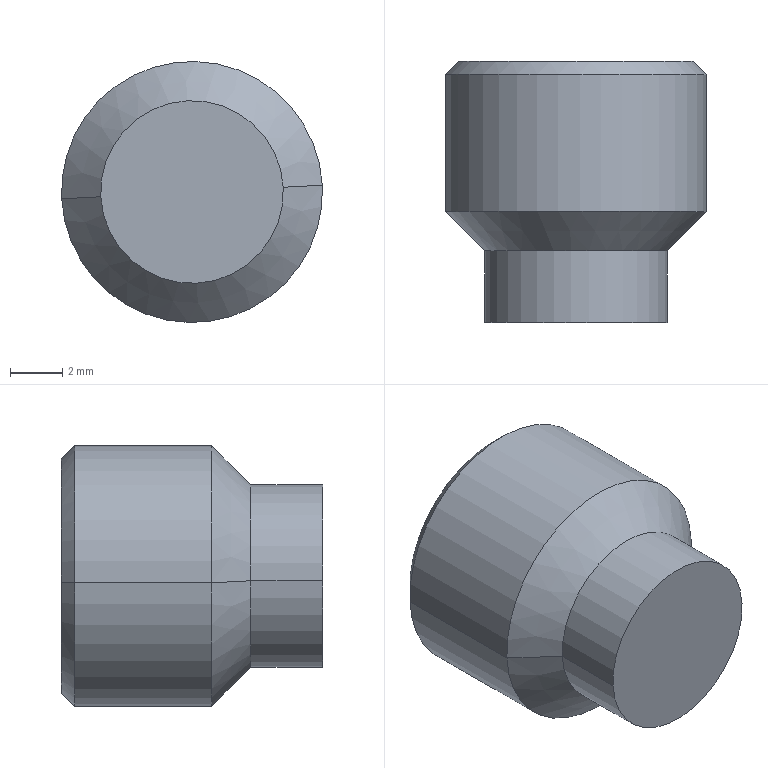Component | SolidWorks | 4-12-12ClampingAxisAssembly-1_4-12-9HeadlessSetScrew-D10-1 | 1 solid | 30 faces | box 10 x 10 x 10 mm | volume 559 mm3 | plane 18 | cone 6 | cylinder 6 | commonest cylinder face diameters 7 x2 5 x2 10 x2
build123d program:
from build123d import *

# Parameters (mm, degrees)
SKETCH1_R            = 2.463
BASE_EXTRUDE_DEPTH   = 20
LPATTERN1_COUNT      = 8
LPATTERN1_PITCH      = 1
SKETCH7_W            = 5
SKETCH7_H            = 6
CUT_EXTRUDE2_DEPTH   = 3
SKETCH4_2_R          = 7.956
CUT_EXTRUDE2_2_DEPTH = 27
SKETCH5_2_R          = 5
EXTRUDE1_DEPTH       = 4
CHAMFER1_SIZE        = 0.5


with BuildPart() as part:
    # Sketch1 → Base-Extrude (new body)
    with BuildSketch(Plane.XY):
        Circle(SKETCH1_R)
    extrude(amount=BASE_EXTRUDE_DEPTH)

    # Boss-Sweep1: sweep along a path in Sketch4
    with BuildLine(Plane(origin=(0, 0, 0.5), x_dir=(-1, 0, 0), z_dir=(0, 0, -1))) as boss_sweep1_path:
        CenterArc((0, 0), 2.463, 0, 360)
    # Sketch2 → Boss-Sweep1 (sweep)
    with BuildSketch(Plane(origin=(0, 0, 0), x_dir=(1, 0, 0), z_dir=(0, 1, 0))):
        Polygon((2.463, 0), (3, -0.3103), (3, -0.4353), (2.463, -0.7457), align=None)
    boss_sweep1 = sweep(path=boss_sweep1_path.line)

    # LPattern1: Boss-Sweep1 ×8
    with Locations(*[(0, 0, i * LPATTERN1_PITCH) for i in range(1, LPATTERN1_COUNT)]):
        add(boss_sweep1)

    # Sketch7 → Boss-Revolve2 (revolve)
    with BuildSketch(Plane(origin=(0, 0, 0), x_dir=(1, 0, 0), z_dir=(0, 1, 0))):
        with Locations((2.5, -23)):
            Rectangle(SKETCH7_W, SKETCH7_H)
    revolve(axis=Axis((0, 0, 0), (0, 0, 1)))

    # Sketch8 → Cut-Extrude2 (cut)
    with BuildSketch(Plane.XY.offset(26)):
        Polygon((-1.417, 2.5), (1.417, 2.5), (2.86, 0), (1.417, -2.5), (-1.417, -2.5), (-2.86, 0), align=None)
    extrude(amount=-CUT_EXTRUDE2_DEPTH, mode=Mode.SUBTRACT)

    # Sketch9 → Cut-Revolve1 (revolve, cut)
    with BuildSketch(Plane(origin=(0, 0, 0), x_dir=(1, 0, 0), z_dir=(0, 1, 0))):
        Polygon((0, -23), (2.5, -23), (2.5, -22.4), (0, -21.73), align=None)
    revolve(axis=Axis((0, 0, 0), (0, 0, 1)), mode=Mode.SUBTRACT)

    # Sketch4_2 → Cut-Extrude2_2 (cut)
    with BuildSketch(Plane(origin=(0, 0, 17.25), x_dir=(-1, 0, 0), z_dir=(0, 0, -1))):
        Circle(SKETCH4_2_R)
    extrude(amount=CUT_EXTRUDE2_2_DEPTH, mode=Mode.SUBTRACT)

    # Sketch5_2 → Extrude1 (add)
    with BuildSketch(Plane(origin=(0, 0, 20), x_dir=(-1, 0, 0), z_dir=(0, 0, -1))):
        Circle(SKETCH5_2_R)
    extrude(amount=EXTRUDE1_DEPTH)

    # Sketch7_2 → Cut-Revolve1_2 (revolve, cut)
    with BuildSketch(Plane(origin=(0, 0, 0), x_dir=(1, 0, 0), z_dir=(0, 1, 0)), mode=Mode.PRIVATE) as cut_revolve1_2_sk:
        Polygon((3.5, -16), (3.5, -18.75), (5, -20.25), (5, -16), align=None)
    revolve(cut_revolve1_2_sk.sketch.rotate(Axis((0, 0, 26), (0, 0, -1)), 180), axis=Axis((0, 0, 26), (0, 0, -1)), mode=Mode.SUBTRACT)

    # Chamfer1
    chamfer1_edges = [part.edges().sort_by_distance(p)[0] for p in [
        (-5, 0, 26),
    ]]
    chamfer(chamfer1_edges, length=CHAMFER1_SIZE)


solid = part.part

# Placed as in the assembly
solid = solid.moved(Location((-19.809, 9.85, 0), (-90, 0, 177)))
STEP:
#1=COLOUR_RGB('',0.7922,0.8196,0.9333);
#2=FILL_AREA_STYLE_COLOUR('',#1);
#3=FILL_AREA_STYLE('',(#2));
#4=SURFACE_STYLE_FILL_AREA(#3);
#5=SURFACE_SIDE_STYLE('',(#4));
#6=SURFACE_STYLE_USAGE(.BOTH.,#5);
#7=PRESENTATION_STYLE_ASSIGNMENT((#6));
#8=CARTESIAN_POINT('',(-0.603,1.411,0.009272));
#9=VERTEX_POINT('',#8);
#10=CARTESIAN_POINT('',(-0.9568,1.411,-0.009272));
#11=VERTEX_POINT('',#10);
#12=CARTESIAN_POINT('',(-0.7799,1.411,0.));
#13=DIRECTION('',(-0.,1.,-0.));
#14=DIRECTION('',(0.9986,0.,0.05234));
#15=AXIS2_PLACEMENT_3D('',#12,#13,#14);
#16=CIRCLE('',#15,0.1772);
#17=EDGE_CURVE('',#9,#11,#16,.T.);
#18=ORIENTED_EDGE('',*,*,#17,.F.);
#19=CARTESIAN_POINT('',(-0.5833,1.392,0.0103));
#20=VERTEX_POINT('',#19);
#21=CARTESIAN_POINT('',(-0.5833,1.392,0.0103));
#22=DIRECTION('',(0.7061,-0.7071,0.03701));
#23=VECTOR('',#22,39.37);
#24=LINE('',#21,#23);
#25=EDGE_CURVE('',#9,#20,#24,.T.);
#26=ORIENTED_EDGE('',*,*,#25,.T.);
#27=CARTESIAN_POINT('',(-0.9765,1.392,-0.0103));
#28=VERTEX_POINT('',#27);
#29=CARTESIAN_POINT('',(-0.7799,1.392,0.));
#30=DIRECTION('',(0.,-1.,0.));
#31=DIRECTION('',(0.9986,0.,0.05234));
#32=AXIS2_PLACEMENT_3D('',#29,#30,#31);
#33=CIRCLE('',#32,0.1969);
#34=EDGE_CURVE('',#28,#20,#33,.T.);
#35=ORIENTED_EDGE('',*,*,#34,.F.);
#36=CARTESIAN_POINT('',(-0.9765,1.392,-0.0103));
#37=DIRECTION('',(-0.7061,-0.7071,-0.03701));
#38=VECTOR('',#37,39.37);
#39=LINE('',#36,#38);
#40=EDGE_CURVE('',#11,#28,#39,.T.);
#41=ORIENTED_EDGE('',*,*,#40,.F.);
#42=EDGE_LOOP('',(#18,#26,#35,#41));
#43=FACE_OUTER_BOUND('',#42,.T.);
#44=CARTESIAN_POINT('',(-0.7799,1.392,0.));
#45=DIRECTION('',(0.,-1.,0.));
#46=DIRECTION('',(-0.9986,0.,-0.05234));
#47=AXIS2_PLACEMENT_3D('',#44,#45,#46);
#48=CONICAL_SURFACE('',#47,0.1969,0.7854);
#49=ADVANCED_FACE('',(#43),#48,.T.);
#50=CARTESIAN_POINT('',(-0.6423,1.018,0.007212));
#51=VERTEX_POINT('',#50);
#52=CARTESIAN_POINT('',(-0.9175,1.018,-0.007212));
#53=VERTEX_POINT('',#52);
#54=CARTESIAN_POINT('',(-0.7799,1.018,0.));
#55=DIRECTION('',(-0.,1.,-0.));
#56=DIRECTION('',(0.9986,0.,0.05234));
#57=AXIS2_PLACEMENT_3D('',#54,#55,#56);
#58=CIRCLE('',#57,0.1378);
#59=EDGE_CURVE('',#51,#53,#58,.T.);
#60=ORIENTED_EDGE('',*,*,#59,.T.);
#61=CARTESIAN_POINT('',(-0.9175,1.126,-0.007212));
#62=VERTEX_POINT('',#61);
#63=CARTESIAN_POINT('',(-0.9175,1.411,-0.007212));
#64=DIRECTION('',(-0.,1.,-0.));
#65=VECTOR('',#64,39.37);
#66=LINE('',#63,#65);
#67=EDGE_CURVE('',#53,#62,#66,.T.);
#68=ORIENTED_EDGE('',*,*,#67,.T.);
#69=CARTESIAN_POINT('',(-0.6423,1.126,0.007212));
#70=VERTEX_POINT('',#69);
#71=CARTESIAN_POINT('',(-0.7799,1.126,0.));
#72=DIRECTION('',(-0.,1.,-0.));
#73=DIRECTION('',(0.9986,0.,0.05234));
#74=AXIS2_PLACEMENT_3D('',#71,#72,#73);
#75=CIRCLE('',#74,0.1378);
#76=EDGE_CURVE('',#70,#62,#75,.T.);
#77=ORIENTED_EDGE('',*,*,#76,.F.);
#78=CARTESIAN_POINT('',(-0.6423,1.411,0.007212));
#79=DIRECTION('',(-0.,1.,-0.));
#80=VECTOR('',#79,39.37);
#81=LINE('',#78,#80);
#82=EDGE_CURVE('',#51,#70,#81,.T.);
#83=ORIENTED_EDGE('',*,*,#82,.F.);
#84=EDGE_LOOP('',(#60,#68,#77,#83));
#85=FACE_OUTER_BOUND('',#84,.T.);
#86=CARTESIAN_POINT('',(-0.7799,1.411,0.));
#87=DIRECTION('',(-0.,1.,-0.));
#88=DIRECTION('',(0.9986,0.,0.05234));
#89=AXIS2_PLACEMENT_3D('',#86,#87,#88);
#90=CYLINDRICAL_SURFACE('',#89,0.1378);
#91=ADVANCED_FACE('',(#85),#90,.T.);
#92=ORIENTED_EDGE('',*,*,#76,.T.);
#93=CARTESIAN_POINT('',(-0.9765,1.185,-0.0103));
#94=VERTEX_POINT('',#93);
#95=CARTESIAN_POINT('',(-0.9175,1.126,-0.007212));
#96=DIRECTION('',(-0.7061,0.7071,-0.03701));
#97=VECTOR('',#96,39.37);
#98=LINE('',#95,#97);
#99=EDGE_CURVE('',#62,#94,#98,.T.);
#100=ORIENTED_EDGE('',*,*,#99,.T.);
#101=CARTESIAN_POINT('',(-0.5833,1.185,0.0103));
#102=VERTEX_POINT('',#101);
#103=CARTESIAN_POINT('',(-0.7799,1.185,0.));
#104=DIRECTION('',(-0.,1.,-0.));
#105=DIRECTION('',(0.9986,0.,0.05234));
#106=AXIS2_PLACEMENT_3D('',#103,#104,#105);
#107=CIRCLE('',#106,0.1969);
#108=EDGE_CURVE('',#102,#94,#107,.T.);
#109=ORIENTED_EDGE('',*,*,#108,.F.);
#110=CARTESIAN_POINT('',(-0.6423,1.126,0.007212));
#111=DIRECTION('',(0.7061,0.7071,0.03701));
#112=VECTOR('',#111,39.37);
#113=LINE('',#110,#112);
#114=EDGE_CURVE('',#70,#102,#113,.T.);
#115=ORIENTED_EDGE('',*,*,#114,.F.);
#116=EDGE_LOOP('',(#92,#100,#109,#115));
#117=FACE_OUTER_BOUND('',#116,.T.);
#118=CARTESIAN_POINT('',(-0.7799,1.126,0.));
#119=DIRECTION('',(-0.,1.,-0.));
#120=DIRECTION('',(0.9986,0.,0.05234));
#121=AXIS2_PLACEMENT_3D('',#118,#119,#120);
#122=CONICAL_SURFACE('',#121,0.1378,0.7854);
#123=ADVANCED_FACE('',(#117),#122,.T.);
#124=CARTESIAN_POINT('',(-0.7799,1.243,0.));
#125=VERTEX_POINT('',#124);
#126=CARTESIAN_POINT('',(-0.6816,1.27,0.005151));
#127=VERTEX_POINT('',#126);
#128=CARTESIAN_POINT('',(-0.6816,1.27,0.005151));
#129=DIRECTION('',(0.9646,0.2588,0.05055));
#130=VECTOR('',#129,39.37);
#131=LINE('',#128,#130);
#132=EDGE_CURVE('',#125,#127,#131,.T.);
#133=ORIENTED_EDGE('',*,*,#132,.F.);
#134=CARTESIAN_POINT('',(-0.8782,1.27,-0.005151));
#135=VERTEX_POINT('',#134);
#136=CARTESIAN_POINT('',(-0.8782,1.27,-0.005151));
#137=DIRECTION('',(-0.9646,0.2588,-0.05055));
#138=VECTOR('',#137,39.37);
#139=LINE('',#136,#138);
#140=EDGE_CURVE('',#125,#135,#139,.T.);
#141=ORIENTED_EDGE('',*,*,#140,.T.);
#142=CARTESIAN_POINT('',(-0.7799,1.27,0.));
#143=DIRECTION('',(0.,-1.,0.));
#144=DIRECTION('',(-0.9986,0.,-0.05234));
#145=AXIS2_PLACEMENT_3D('',#142,#143,#144);
#146=CIRCLE('',#145,0.09843);
#147=EDGE_CURVE('',#127,#135,#146,.T.);
#148=ORIENTED_EDGE('',*,*,#147,.F.);
#149=EDGE_LOOP('',(#133,#141,#148));
#150=FACE_OUTER_BOUND('',#149,.T.);
#151=CARTESIAN_POINT('',(-0.7799,1.27,0.));
#152=DIRECTION('',(-0.,1.,-0.));
#153=DIRECTION('',(0.9986,0.,0.05234));
#154=AXIS2_PLACEMENT_3D('',#151,#152,#153);
#155=CONICAL_SURFACE('',#154,0.09843,1.309);
#156=ADVANCED_FACE('',(#150),#155,.F.);
#157=CARTESIAN_POINT('',(-0.6816,1.293,0.005151));
#158=VERTEX_POINT('',#157);
#159=CARTESIAN_POINT('',(-0.6908,1.293,0.0419));
#160=VERTEX_POINT('',#159);
#161=CARTESIAN_POINT('',(-0.7799,1.293,0.));
#162=DIRECTION('',(0.,-1.,0.));
#163=DIRECTION('',(0.9986,0.,0.05234));
#164=AXIS2_PLACEMENT_3D('',#161,#162,#163);
#165=CIRCLE('',#164,0.09843);
#166=EDGE_CURVE('',#158,#160,#165,.T.);
#167=ORIENTED_EDGE('',*,*,#166,.F.);
#168=CARTESIAN_POINT('',(-0.6816,0.3878,0.005151));
#169=DIRECTION('',(0.,-1.,0.));
#170=VECTOR('',#169,39.37);
#171=LINE('',#168,#170);
#172=EDGE_CURVE('',#158,#127,#171,.T.);
#173=ORIENTED_EDGE('',*,*,#172,.T.);
#174=ORIENTED_EDGE('',*,*,#147,.T.);
#175=CARTESIAN_POINT('',(-0.8782,1.293,-0.005151));
#176=VERTEX_POINT('',#175);
#177=CARTESIAN_POINT('',(-0.8782,0.3878,-0.005151));
#178=DIRECTION('',(0.,-1.,0.));
#179=VECTOR('',#178,39.37);
#180=LINE('',#177,#179);
#181=EDGE_CURVE('',#176,#135,#180,.T.);
#182=ORIENTED_EDGE('',*,*,#181,.F.);
#183=CARTESIAN_POINT('',(-0.8728,1.293,0.03236));
#184=VERTEX_POINT('',#183);
#185=CARTESIAN_POINT('',(-0.7799,1.293,0.));
#186=DIRECTION('',(0.,-1.,0.));
#187=DIRECTION('',(0.9986,0.,0.05234));
#188=AXIS2_PLACEMENT_3D('',#185,#186,#187);
#189=CIRCLE('',#188,0.09843);
#190=EDGE_CURVE('',#184,#176,#189,.T.);
#191=ORIENTED_EDGE('',*,*,#190,.F.);
#192=CARTESIAN_POINT('',(-0.8607,1.293,0.05618));
#193=VERTEX_POINT('',#192);
#194=CARTESIAN_POINT('',(-0.7799,1.293,0.));
#195=DIRECTION('',(0.,-1.,0.));
#196=DIRECTION('',(-0.9986,0.,-0.05234));
#197=AXIS2_PLACEMENT_3D('',#194,#195,#196);
#198=CIRCLE('',#197,0.09843);
#199=EDGE_CURVE('',#193,#184,#198,.T.);
#200=ORIENTED_EDGE('',*,*,#199,.F.);
#201=CARTESIAN_POINT('',(-0.785,1.293,0.09829));
#202=VERTEX_POINT('',#201);
#203=CARTESIAN_POINT('',(-0.7799,1.293,0.));
#204=DIRECTION('',(0.,-1.,0.));
#205=DIRECTION('',(0.9986,0.,0.05234));
#206=AXIS2_PLACEMENT_3D('',#203,#204,#205);
#207=CIRCLE('',#206,0.09843);
#208=EDGE_CURVE('',#202,#193,#207,.T.);
#209=ORIENTED_EDGE('',*,*,#208,.F.);
#210=CARTESIAN_POINT('',(-0.7054,1.293,0.06432));
#211=VERTEX_POINT('',#210);
#212=CARTESIAN_POINT('',(-0.7799,1.293,0.));
#213=DIRECTION('',(0.,-1.,0.));
#214=DIRECTION('',(0.9986,0.,0.05234));
#215=AXIS2_PLACEMENT_3D('',#212,#213,#214);
#216=CIRCLE('',#215,0.09843);
#217=EDGE_CURVE('',#211,#202,#216,.T.);
#218=ORIENTED_EDGE('',*,*,#217,.F.);
#219=CARTESIAN_POINT('',(-0.7799,1.293,0.));
#220=DIRECTION('',(0.,-1.,0.));
#221=DIRECTION('',(-0.9986,0.,-0.05234));
#222=AXIS2_PLACEMENT_3D('',#219,#220,#221);
#223=CIRCLE('',#222,0.09843);
#224=EDGE_CURVE('',#160,#211,#223,.T.);
#225=ORIENTED_EDGE('',*,*,#224,.F.);
#226=EDGE_LOOP('',(#167,#173,#174,#182,#191,#200,#209,#218,#225));
#227=FACE_OUTER_BOUND('',#226,.T.);
#228=CARTESIAN_POINT('',(-0.7799,0.3878,0.));
#229=DIRECTION('',(0.,-1.,0.));
#230=DIRECTION('',(-0.9986,0.,-0.05234));
#231=AXIS2_PLACEMENT_3D('',#228,#229,#230);
#232=CYLINDRICAL_SURFACE('',#231,0.09843);
#233=ADVANCED_FACE('',(#227),#232,.F.);
#234=ORIENTED_EDGE('',*,*,#34,.T.);
#235=CARTESIAN_POINT('',(-0.5833,0.3878,0.0103));
#236=DIRECTION('',(0.,-1.,0.));
#237=VECTOR('',#236,39.37);
#238=LINE('',#235,#237);
#239=EDGE_CURVE('',#20,#102,#238,.T.);
#240=ORIENTED_EDGE('',*,*,#239,.T.);
#241=ORIENTED_EDGE('',*,*,#108,.T.);
#242=CARTESIAN_POINT('',(-0.9765,0.3878,-0.0103));
#243=DIRECTION('',(0.,-1.,0.));
#244=VECTOR('',#243,39.37);
#245=LINE('',#242,#244);
#246=EDGE_CURVE('',#28,#94,#245,.T.);
#247=ORIENTED_EDGE('',*,*,#246,.F.);
#248=EDGE_LOOP('',(#234,#240,#241,#247));
#249=FACE_OUTER_BOUND('',#248,.T.);
#250=CARTESIAN_POINT('',(-0.7799,0.3878,0.));
#251=DIRECTION('',(0.,-1.,0.));
#252=DIRECTION('',(-0.9986,0.,-0.05234));
#253=AXIS2_PLACEMENT_3D('',#250,#251,#252);
#254=CYLINDRICAL_SURFACE('',#253,0.1969);
#255=ADVANCED_FACE('',(#249),#254,.T.);
#256=CARTESIAN_POINT('',(-0.7293,1.293,0.1012));
#257=VERTEX_POINT('',#256);
#258=CARTESIAN_POINT('',(-0.7293,1.293,0.1012));
#259=DIRECTION('',(0.5446,0.,-0.8387));
#260=VECTOR('',#259,39.37);
#261=LINE('',#258,#260);
#262=EDGE_CURVE('',#257,#211,#261,.T.);
#263=ORIENTED_EDGE('',*,*,#262,.T.);
#264=ORIENTED_EDGE('',*,*,#217,.T.);
#265=CARTESIAN_POINT('',(-0.8407,1.293,0.09537));
#266=DIRECTION('',(0.9986,0.,0.05234));
#267=VECTOR('',#266,39.37);
#268=LINE('',#265,#267);
#269=EDGE_CURVE('',#202,#257,#268,.T.);
#270=ORIENTED_EDGE('',*,*,#269,.T.);
#271=EDGE_LOOP('',(#263,#264,#270));
#272=FACE_OUTER_BOUND('',#271,.T.);
#273=CARTESIAN_POINT('',(-0.7697,1.293,-0.1948));
#274=DIRECTION('',(-0.,1.,-0.));
#275=DIRECTION('',(0.9986,0.,0.05234));
#276=AXIS2_PLACEMENT_3D('',#273,#274,#275);
#277=PLANE('',#276);
#278=ADVANCED_FACE('',(#272),#277,.T.);
#279=CARTESIAN_POINT('',(-0.8407,1.293,0.09537));
#280=VERTEX_POINT('',#279);
#281=CARTESIAN_POINT('',(-0.8407,1.293,0.09537));
#282=DIRECTION('',(0.9986,0.,0.05234));
#283=VECTOR('',#282,39.37);
#284=LINE('',#281,#283);
#285=EDGE_CURVE('',#280,#202,#284,.T.);
#286=ORIENTED_EDGE('',*,*,#285,.T.);
#287=ORIENTED_EDGE('',*,*,#208,.T.);
#288=CARTESIAN_POINT('',(-0.8407,1.293,0.09537));
#289=DIRECTION('',(-0.454,-0.,-0.891));
#290=VECTOR('',#289,39.37);
#291=LINE('',#288,#290);
#292=EDGE_CURVE('',#280,#193,#291,.T.);
#293=ORIENTED_EDGE('',*,*,#292,.F.);
#294=EDGE_LOOP('',(#286,#287,#293));
#295=FACE_OUTER_BOUND('',#294,.T.);
#296=CARTESIAN_POINT('',(-0.7697,1.293,-0.1948));
#297=DIRECTION('',(-0.,1.,-0.));
#298=DIRECTION('',(0.9986,0.,0.05234));
#299=AXIS2_PLACEMENT_3D('',#296,#297,#298);
#300=PLANE('',#299);
#301=ADVANCED_FACE('',(#295),#300,.T.);
#302=CARTESIAN_POINT('',(-0.8923,1.293,-0.005893));
#303=VERTEX_POINT('',#302);
#304=CARTESIAN_POINT('',(-0.8407,1.293,0.09537));
#305=DIRECTION('',(-0.454,-0.,-0.891));
#306=VECTOR('',#305,39.37);
#307=LINE('',#304,#306);
#308=EDGE_CURVE('',#184,#303,#307,.T.);
#309=ORIENTED_EDGE('',*,*,#308,.F.);
#310=ORIENTED_EDGE('',*,*,#190,.T.);
#311=CARTESIAN_POINT('',(-0.8689,1.293,-0.0419));
#312=VERTEX_POINT('',#311);
#313=CARTESIAN_POINT('',(-0.7799,1.293,0.));
#314=DIRECTION('',(0.,-1.,0.));
#315=DIRECTION('',(0.9986,0.,0.05234));
#316=AXIS2_PLACEMENT_3D('',#313,#314,#315);
#317=CIRCLE('',#316,0.09843);
#318=EDGE_CURVE('',#176,#312,#317,.T.);
#319=ORIENTED_EDGE('',*,*,#318,.T.);
#320=CARTESIAN_POINT('',(-0.8304,1.293,-0.1012));
#321=DIRECTION('',(-0.5446,-0.,0.8387));
#322=VECTOR('',#321,39.37);
#323=LINE('',#320,#322);
#324=EDGE_CURVE('',#312,#303,#323,.T.);
#325=ORIENTED_EDGE('',*,*,#324,.T.);
#326=EDGE_LOOP('',(#309,#310,#319,#325));
#327=FACE_OUTER_BOUND('',#326,.T.);
#328=CARTESIAN_POINT('',(-0.7697,1.293,-0.1948));
#329=DIRECTION('',(-0.,1.,-0.));
#330=DIRECTION('',(0.9986,0.,0.05234));
#331=AXIS2_PLACEMENT_3D('',#328,#329,#330);
#332=PLANE('',#331);
#333=ADVANCED_FACE('',(#327),#332,.T.);
#334=CARTESIAN_POINT('',(-0.8304,1.293,-0.1012));
#335=VERTEX_POINT('',#334);
#336=CARTESIAN_POINT('',(-0.8544,1.293,-0.06432));
#337=VERTEX_POINT('',#336);
#338=CARTESIAN_POINT('',(-0.8304,1.293,-0.1012));
#339=DIRECTION('',(-0.5446,-0.,0.8387));
#340=VECTOR('',#339,39.37);
#341=LINE('',#338,#340);
#342=EDGE_CURVE('',#335,#337,#341,.T.);
#343=ORIENTED_EDGE('',*,*,#342,.T.);
#344=CARTESIAN_POINT('',(-0.7747,1.293,-0.09829));
#345=VERTEX_POINT('',#344);
#346=CARTESIAN_POINT('',(-0.7799,1.293,0.));
#347=DIRECTION('',(0.,-1.,0.));
#348=DIRECTION('',(0.9986,0.,0.05234));
#349=AXIS2_PLACEMENT_3D('',#346,#347,#348);
#350=CIRCLE('',#349,0.09843);
#351=EDGE_CURVE('',#337,#345,#350,.T.);
#352=ORIENTED_EDGE('',*,*,#351,.T.);
#353=CARTESIAN_POINT('',(-0.8304,1.293,-0.1012));
#354=DIRECTION('',(0.9986,0.,0.05234));
#355=VECTOR('',#354,39.37);
#356=LINE('',#353,#355);
#357=EDGE_CURVE('',#335,#345,#356,.T.);
#358=ORIENTED_EDGE('',*,*,#357,.F.);
#359=EDGE_LOOP('',(#343,#352,#358));
#360=FACE_OUTER_BOUND('',#359,.T.);
#361=CARTESIAN_POINT('',(-0.7697,1.293,-0.1948));
#362=DIRECTION('',(-0.,1.,-0.));
#363=DIRECTION('',(0.9986,0.,0.05234));
#364=AXIS2_PLACEMENT_3D('',#361,#362,#363);
#365=PLANE('',#364);
#366=ADVANCED_FACE('',(#360),#365,.T.);
#367=CARTESIAN_POINT('',(-0.719,1.293,-0.09537));
#368=VERTEX_POINT('',#367);
#369=CARTESIAN_POINT('',(-0.8304,1.293,-0.1012));
#370=DIRECTION('',(0.9986,0.,0.05234));
#371=VECTOR('',#370,39.37);
#372=LINE('',#369,#371);
#373=EDGE_CURVE('',#345,#368,#372,.T.);
#374=ORIENTED_EDGE('',*,*,#373,.F.);
#375=CARTESIAN_POINT('',(-0.6991,1.293,-0.05618));
#376=VERTEX_POINT('',#375);
#377=CARTESIAN_POINT('',(-0.7799,1.293,0.));
#378=DIRECTION('',(0.,-1.,0.));
#379=DIRECTION('',(0.9986,0.,0.05234));
#380=AXIS2_PLACEMENT_3D('',#377,#378,#379);
#381=CIRCLE('',#380,0.09843);
#382=EDGE_CURVE('',#345,#376,#381,.T.);
#383=ORIENTED_EDGE('',*,*,#382,.T.);
#384=CARTESIAN_POINT('',(-0.719,1.293,-0.09537));
#385=DIRECTION('',(0.454,0.,0.891));
#386=VECTOR('',#385,39.37);
#387=LINE('',#384,#386);
#388=EDGE_CURVE('',#368,#376,#387,.T.);
#389=ORIENTED_EDGE('',*,*,#388,.F.);
#390=EDGE_LOOP('',(#374,#383,#389));
#391=FACE_OUTER_BOUND('',#390,.T.);
#392=CARTESIAN_POINT('',(-0.7697,1.293,-0.1948));
#393=DIRECTION('',(-0.,1.,-0.));
#394=DIRECTION('',(0.9986,0.,0.05234));
#395=AXIS2_PLACEMENT_3D('',#392,#393,#394);
#396=PLANE('',#395);
#397=ADVANCED_FACE('',(#391),#396,.T.);
#398=ORIENTED_EDGE('',*,*,#239,.F.);
#399=CARTESIAN_POINT('',(-0.7799,1.392,0.));
#400=DIRECTION('',(0.,-1.,0.));
#401=DIRECTION('',(0.9986,0.,0.05234));
#402=AXIS2_PLACEMENT_3D('',#399,#400,#401);
#403=CIRCLE('',#402,0.1969);
#404=EDGE_CURVE('',#20,#28,#403,.T.);
#405=ORIENTED_EDGE('',*,*,#404,.T.);
#406=ORIENTED_EDGE('',*,*,#246,.T.);
#407=CARTESIAN_POINT('',(-0.7799,1.185,0.));
#408=DIRECTION('',(-0.,1.,-0.));
#409=DIRECTION('',(0.9986,0.,0.05234));
#410=AXIS2_PLACEMENT_3D('',#407,#408,#409);
#411=CIRCLE('',#410,0.1969);
#412=EDGE_CURVE('',#94,#102,#411,.T.);
#413=ORIENTED_EDGE('',*,*,#412,.T.);
#414=EDGE_LOOP('',(#398,#405,#406,#413));
#415=FACE_OUTER_BOUND('',#414,.T.);
#416=CARTESIAN_POINT('',(-0.7799,0.3878,0.));
#417=DIRECTION('',(0.,-1.,0.));
#418=DIRECTION('',(-0.9986,0.,-0.05234));
#419=AXIS2_PLACEMENT_3D('',#416,#417,#418);
#420=CYLINDRICAL_SURFACE('',#419,0.1969);
#421=ADVANCED_FACE('',(#415),#420,.T.);
#422=CARTESIAN_POINT('',(-0.7799,1.411,0.));
#423=DIRECTION('',(-0.,1.,-0.));
#424=DIRECTION('',(0.9986,0.,0.05234));
#425=AXIS2_PLACEMENT_3D('',#422,#423,#424);
#426=CIRCLE('',#425,0.1772);
#427=EDGE_CURVE('',#11,#9,#426,.T.);
#428=ORIENTED_EDGE('',*,*,#427,.T.);
#429=ORIENTED_EDGE('',*,*,#17,.T.);
#430=EDGE_LOOP('',(#428,#429));
#431=FACE_OUTER_BOUND('',#430,.T.);
#432=CARTESIAN_POINT('',(-0.8304,1.411,-0.1012));
#433=VERTEX_POINT('',#432);
#434=CARTESIAN_POINT('',(-0.8923,1.411,-0.005893));
#435=VERTEX_POINT('',#434);
#436=CARTESIAN_POINT('',(-0.8304,1.411,-0.1012));
#437=DIRECTION('',(-0.5446,-0.,0.8387));
#438=VECTOR('',#437,39.37);
#439=LINE('',#436,#438);
#440=EDGE_CURVE('',#433,#435,#439,.T.);
#441=ORIENTED_EDGE('',*,*,#440,.F.);
#442=CARTESIAN_POINT('',(-0.719,1.411,-0.09537));
#443=VERTEX_POINT('',#442);
#444=CARTESIAN_POINT('',(-0.8304,1.411,-0.1012));
#445=DIRECTION('',(0.9986,0.,0.05234));
#446=VECTOR('',#445,39.37);
#447=LINE('',#444,#446);
#448=EDGE_CURVE('',#433,#443,#447,.T.);
#449=ORIENTED_EDGE('',*,*,#448,.T.);
#450=CARTESIAN_POINT('',(-0.6674,1.411,0.005893));
#451=VERTEX_POINT('',#450);
#452=CARTESIAN_POINT('',(-0.719,1.411,-0.09537));
#453=DIRECTION('',(0.454,0.,0.891));
#454=VECTOR('',#453,39.37);
#455=LINE('',#452,#454);
#456=EDGE_CURVE('',#443,#451,#455,.T.);
#457=ORIENTED_EDGE('',*,*,#456,.T.);
#458=CARTESIAN_POINT('',(-0.7293,1.411,0.1012));
#459=VERTEX_POINT('',#458);
#460=CARTESIAN_POINT('',(-0.7293,1.411,0.1012));
#461=DIRECTION('',(0.5446,0.,-0.8387));
#462=VECTOR('',#461,39.37);
#463=LINE('',#460,#462);
#464=EDGE_CURVE('',#459,#451,#463,.T.);
#465=ORIENTED_EDGE('',*,*,#464,.F.);
#466=CARTESIAN_POINT('',(-0.8407,1.411,0.09537));
#467=VERTEX_POINT('',#466);
#468=CARTESIAN_POINT('',(-0.8407,1.411,0.09537));
#469=DIRECTION('',(0.9986,0.,0.05234));
#470=VECTOR('',#469,39.37);
#471=LINE('',#468,#470);
#472=EDGE_CURVE('',#467,#459,#471,.T.);
#473=ORIENTED_EDGE('',*,*,#472,.F.);
#474=CARTESIAN_POINT('',(-0.8407,1.411,0.09537));
#475=DIRECTION('',(-0.454,-0.,-0.891));
#476=VECTOR('',#475,39.37);
#477=LINE('',#474,#476);
#478=EDGE_CURVE('',#467,#435,#477,.T.);
#479=ORIENTED_EDGE('',*,*,#478,.T.);
#480=EDGE_LOOP('',(#441,#449,#457,#465,#473,#479));
#481=FACE_BOUND('',#480,.T.);
#482=CARTESIAN_POINT('',(-0.5833,1.411,0.0103));
#483=DIRECTION('',(-0.,1.,-0.));
#484=DIRECTION('',(0.9986,0.,0.05234));
#485=AXIS2_PLACEMENT_3D('',#482,#483,#484);
#486=PLANE('',#485);
#487=ADVANCED_FACE('',(#431,#481),#486,.T.);
#488=ORIENTED_EDGE('',*,*,#440,.T.);
#489=CARTESIAN_POINT('',(-0.8923,1.293,-0.005893));
#490=DIRECTION('',(-0.,1.,-0.));
#491=VECTOR('',#490,39.37);
#492=LINE('',#489,#491);
#493=EDGE_CURVE('',#303,#435,#492,.T.);
#494=ORIENTED_EDGE('',*,*,#493,.F.);
#495=ORIENTED_EDGE('',*,*,#324,.F.);
#496=CARTESIAN_POINT('',(-0.8304,1.293,-0.1012));
#497=DIRECTION('',(-0.5446,-0.,0.8387));
#498=VECTOR('',#497,39.37);
#499=LINE('',#496,#498);
#500=EDGE_CURVE('',#337,#312,#499,.T.);
#501=ORIENTED_EDGE('',*,*,#500,.F.);
#502=ORIENTED_EDGE('',*,*,#342,.F.);
#503=CARTESIAN_POINT('',(-0.8304,1.293,-0.1012));
#504=DIRECTION('',(-0.,1.,-0.));
#505=VECTOR('',#504,39.37);
#506=LINE('',#503,#505);
#507=EDGE_CURVE('',#335,#433,#506,.T.);
#508=ORIENTED_EDGE('',*,*,#507,.T.);
#509=EDGE_LOOP('',(#488,#494,#495,#501,#502,#508));
#510=FACE_OUTER_BOUND('',#509,.T.);
#511=CARTESIAN_POINT('',(-0.8304,1.293,-0.1012));
#512=DIRECTION('',(-0.8387,-0.,-0.5446));
#513=DIRECTION('',(-0.5446,-0.,0.8387));
#514=AXIS2_PLACEMENT_3D('',#511,#512,#513);
#515=PLANE('',#514);
#516=ADVANCED_FACE('',(#510),#515,.F.);
#517=ORIENTED_EDGE('',*,*,#448,.F.);
#518=ORIENTED_EDGE('',*,*,#507,.F.);
#519=ORIENTED_EDGE('',*,*,#357,.T.);
#520=ORIENTED_EDGE('',*,*,#373,.T.);
#521=CARTESIAN_POINT('',(-0.719,1.293,-0.09537));
#522=DIRECTION('',(-0.,1.,-0.));
#523=VECTOR('',#522,39.37);
#524=LINE('',#521,#523);
#525=EDGE_CURVE('',#368,#443,#524,.T.);
#526=ORIENTED_EDGE('',*,*,#525,.T.);
#527=EDGE_LOOP('',(#517,#518,#519,#520,#526));
#528=FACE_OUTER_BOUND('',#527,.T.);
#529=CARTESIAN_POINT('',(-0.8304,1.293,-0.1012));
#530=DIRECTION('',(-0.05234,0.,0.9986));
#531=DIRECTION('',(0.9986,0.,0.05234));
#532=AXIS2_PLACEMENT_3D('',#529,#530,#531);
#533=PLANE('',#532);
#534=ADVANCED_FACE('',(#528),#533,.T.);
#535=ORIENTED_EDGE('',*,*,#456,.F.);
#536=ORIENTED_EDGE('',*,*,#525,.F.);
#537=ORIENTED_EDGE('',*,*,#388,.T.);
#538=CARTESIAN_POINT('',(-0.6869,1.293,-0.03236));
#539=VERTEX_POINT('',#538);
#540=CARTESIAN_POINT('',(-0.719,1.293,-0.09537));
#541=DIRECTION('',(0.454,0.,0.891));
#542=VECTOR('',#541,39.37);
#543=LINE('',#540,#542);
#544=EDGE_CURVE('',#376,#539,#543,.T.);
#545=ORIENTED_EDGE('',*,*,#544,.T.);
#546=CARTESIAN_POINT('',(-0.6674,1.293,0.005893));
#547=VERTEX_POINT('',#546);
#548=CARTESIAN_POINT('',(-0.719,1.293,-0.09537));
#549=DIRECTION('',(0.454,0.,0.891));
#550=VECTOR('',#549,39.37);
#551=LINE('',#548,#550);
#552=EDGE_CURVE('',#539,#547,#551,.T.);
#553=ORIENTED_EDGE('',*,*,#552,.T.);
#554=CARTESIAN_POINT('',(-0.6674,1.293,0.005893));
#555=DIRECTION('',(-0.,1.,-0.));
#556=VECTOR('',#555,39.37);
#557=LINE('',#554,#556);
#558=EDGE_CURVE('',#547,#451,#557,.T.);
#559=ORIENTED_EDGE('',*,*,#558,.T.);
#560=EDGE_LOOP('',(#535,#536,#537,#545,#553,#559));
#561=FACE_OUTER_BOUND('',#560,.T.);
#562=CARTESIAN_POINT('',(-0.719,1.293,-0.09537));
#563=DIRECTION('',(-0.891,-0.,0.454));
#564=DIRECTION('',(0.454,0.,0.891));
#565=AXIS2_PLACEMENT_3D('',#562,#563,#564);
#566=PLANE('',#565);
#567=ADVANCED_FACE('',(#561),#566,.T.);
#568=ORIENTED_EDGE('',*,*,#464,.T.);
#569=ORIENTED_EDGE('',*,*,#558,.F.);
#570=CARTESIAN_POINT('',(-0.7293,1.293,0.1012));
#571=DIRECTION('',(0.5446,0.,-0.8387));
#572=VECTOR('',#571,39.37);
#573=LINE('',#570,#572);
#574=EDGE_CURVE('',#160,#547,#573,.T.);
#575=ORIENTED_EDGE('',*,*,#574,.F.);
#576=CARTESIAN_POINT('',(-0.7293,1.293,0.1012));
#577=DIRECTION('',(0.5446,0.,-0.8387));
#578=VECTOR('',#577,39.37);
#579=LINE('',#576,#578);
#580=EDGE_CURVE('',#211,#160,#579,.T.);
#581=ORIENTED_EDGE('',*,*,#580,.F.);
#582=ORIENTED_EDGE('',*,*,#262,.F.);
#583=CARTESIAN_POINT('',(-0.7293,1.293,0.1012));
#584=DIRECTION('',(-0.,1.,-0.));
#585=VECTOR('',#584,39.37);
#586=LINE('',#583,#585);
#587=EDGE_CURVE('',#257,#459,#586,.T.);
#588=ORIENTED_EDGE('',*,*,#587,.T.);
#589=EDGE_LOOP('',(#568,#569,#575,#581,#582,#588));
#590=FACE_OUTER_BOUND('',#589,.T.);
#591=CARTESIAN_POINT('',(-0.7293,1.293,0.1012));
#592=DIRECTION('',(0.8387,0.,0.5446));
#593=DIRECTION('',(0.5446,0.,-0.8387));
#594=AXIS2_PLACEMENT_3D('',#591,#592,#593);
#595=PLANE('',#594);
#596=ADVANCED_FACE('',(#590),#595,.F.);
#597=ORIENTED_EDGE('',*,*,#472,.T.);
#598=ORIENTED_EDGE('',*,*,#587,.F.);
#599=ORIENTED_EDGE('',*,*,#269,.F.);
#600=ORIENTED_EDGE('',*,*,#285,.F.);
#601=CARTESIAN_POINT('',(-0.8407,1.293,0.09537));
#602=DIRECTION('',(-0.,1.,-0.));
#603=VECTOR('',#602,39.37);
#604=LINE('',#601,#603);
#605=EDGE_CURVE('',#280,#467,#604,.T.);
#606=ORIENTED_EDGE('',*,*,#605,.T.);
#607=EDGE_LOOP('',(#597,#598,#599,#600,#606));
#608=FACE_OUTER_BOUND('',#607,.T.);
#609=CARTESIAN_POINT('',(-0.8407,1.293,0.09537));
#610=DIRECTION('',(-0.05234,0.,0.9986));
#611=DIRECTION('',(0.9986,0.,0.05234));
#612=AXIS2_PLACEMENT_3D('',#609,#610,#611);
#613=PLANE('',#612);
#614=ADVANCED_FACE('',(#608),#613,.F.);
#615=ORIENTED_EDGE('',*,*,#478,.F.);
#616=ORIENTED_EDGE('',*,*,#605,.F.);
#617=ORIENTED_EDGE('',*,*,#292,.T.);
#618=CARTESIAN_POINT('',(-0.8407,1.293,0.09537));
#619=DIRECTION('',(-0.454,-0.,-0.891));
#620=VECTOR('',#619,39.37);
#621=LINE('',#618,#620);
#622=EDGE_CURVE('',#193,#184,#621,.T.);
#623=ORIENTED_EDGE('',*,*,#622,.T.);
#624=ORIENTED_EDGE('',*,*,#308,.T.);
#625=ORIENTED_EDGE('',*,*,#493,.T.);
#626=EDGE_LOOP('',(#615,#616,#617,#623,#624,#625));
#627=FACE_OUTER_BOUND('',#626,.T.);
#628=CARTESIAN_POINT('',(-0.8407,1.293,0.09537));
#629=DIRECTION('',(0.891,0.,-0.454));
#630=DIRECTION('',(-0.454,-0.,-0.891));
#631=AXIS2_PLACEMENT_3D('',#628,#629,#630);
#632=PLANE('',#631);
#633=ADVANCED_FACE('',(#627),#632,.T.);
#634=ORIENTED_EDGE('',*,*,#552,.F.);
#635=CARTESIAN_POINT('',(-0.7799,1.293,0.));
#636=DIRECTION('',(0.,-1.,0.));
#637=DIRECTION('',(0.9986,0.,0.05234));
#638=AXIS2_PLACEMENT_3D('',#635,#636,#637);
#639=CIRCLE('',#638,0.09843);
#640=EDGE_CURVE('',#539,#158,#639,.T.);
#641=ORIENTED_EDGE('',*,*,#640,.T.);
#642=ORIENTED_EDGE('',*,*,#166,.T.);
#643=ORIENTED_EDGE('',*,*,#574,.T.);
#644=EDGE_LOOP('',(#634,#641,#642,#643));
#645=FACE_OUTER_BOUND('',#644,.T.);
#646=CARTESIAN_POINT('',(-0.7697,1.293,-0.1948));
#647=DIRECTION('',(-0.,1.,-0.));
#648=DIRECTION('',(0.9986,0.,0.05234));
#649=AXIS2_PLACEMENT_3D('',#646,#647,#648);
#650=PLANE('',#649);
#651=ADVANCED_FACE('',(#645),#650,.T.);
#652=ORIENTED_EDGE('',*,*,#500,.T.);
#653=CARTESIAN_POINT('',(-0.7799,1.293,0.));
#654=DIRECTION('',(0.,-1.,0.));
#655=DIRECTION('',(-0.9986,0.,-0.05234));
#656=AXIS2_PLACEMENT_3D('',#653,#654,#655);
#657=CIRCLE('',#656,0.09843);
#658=EDGE_CURVE('',#312,#337,#657,.T.);
#659=ORIENTED_EDGE('',*,*,#658,.T.);
#660=EDGE_LOOP('',(#652,#659));
#661=FACE_OUTER_BOUND('',#660,.T.);
#662=CARTESIAN_POINT('',(-0.7799,1.293,0.));
#663=DIRECTION('',(0.,-1.,0.));
#664=DIRECTION('',(-0.9986,-0.,-0.05234));
#665=AXIS2_PLACEMENT_3D('',#662,#663,#664);
#666=PLANE('',#665);
#667=ADVANCED_FACE('',(#661),#666,.T.);
#668=ORIENTED_EDGE('',*,*,#580,.T.);
#669=ORIENTED_EDGE('',*,*,#224,.T.);
#670=EDGE_LOOP('',(#668,#669));
#671=FACE_OUTER_BOUND('',#670,.T.);
#672=CARTESIAN_POINT('',(-0.7799,1.293,0.));
#673=DIRECTION('',(0.,-1.,0.));
#674=DIRECTION('',(-0.9986,-0.,-0.05234));
#675=AXIS2_PLACEMENT_3D('',#672,#673,#674);
#676=PLANE('',#675);
#677=ADVANCED_FACE('',(#671),#676,.T.);
#678=CARTESIAN_POINT('',(-0.7799,1.293,0.));
#679=DIRECTION('',(0.,-1.,0.));
#680=DIRECTION('',(-0.9986,0.,-0.05234));
#681=AXIS2_PLACEMENT_3D('',#678,#679,#680);
#682=CIRCLE('',#681,0.09843);
#683=EDGE_CURVE('',#376,#539,#682,.T.);
#684=ORIENTED_EDGE('',*,*,#683,.T.);
#685=ORIENTED_EDGE('',*,*,#544,.F.);
#686=EDGE_LOOP('',(#684,#685));
#687=FACE_OUTER_BOUND('',#686,.T.);
#688=CARTESIAN_POINT('',(-0.7799,1.293,0.));
#689=DIRECTION('',(0.,-1.,0.));
#690=DIRECTION('',(-0.9986,-0.,-0.05234));
#691=AXIS2_PLACEMENT_3D('',#688,#689,#690);
#692=PLANE('',#691);
#693=ADVANCED_FACE('',(#687),#692,.T.);
#694=ORIENTED_EDGE('',*,*,#199,.T.);
#695=ORIENTED_EDGE('',*,*,#622,.F.);
#696=EDGE_LOOP('',(#694,#695));
#697=FACE_OUTER_BOUND('',#696,.T.);
#698=CARTESIAN_POINT('',(-0.7799,1.293,0.));
#699=DIRECTION('',(0.,-1.,0.));
#700=DIRECTION('',(-0.9986,-0.,-0.05234));
#701=AXIS2_PLACEMENT_3D('',#698,#699,#700);
#702=PLANE('',#701);
#703=ADVANCED_FACE('',(#697),#702,.T.);
#704=ORIENTED_EDGE('',*,*,#172,.F.);
#705=ORIENTED_EDGE('',*,*,#640,.F.);
#706=ORIENTED_EDGE('',*,*,#683,.F.);
#707=ORIENTED_EDGE('',*,*,#382,.F.);
#708=ORIENTED_EDGE('',*,*,#351,.F.);
#709=ORIENTED_EDGE('',*,*,#658,.F.);
#710=ORIENTED_EDGE('',*,*,#318,.F.);
#711=ORIENTED_EDGE('',*,*,#181,.T.);
#712=CARTESIAN_POINT('',(-0.7799,1.27,0.));
#713=DIRECTION('',(0.,-1.,0.));
#714=DIRECTION('',(-0.9986,0.,-0.05234));
#715=AXIS2_PLACEMENT_3D('',#712,#713,#714);
#716=CIRCLE('',#715,0.09843);
#717=EDGE_CURVE('',#135,#127,#716,.T.);
#718=ORIENTED_EDGE('',*,*,#717,.T.);
#719=EDGE_LOOP('',(#704,#705,#706,#707,#708,#709,#710,#711,#718));
#720=FACE_OUTER_BOUND('',#719,.T.);
#721=CARTESIAN_POINT('',(-0.7799,0.3878,0.));
#722=DIRECTION('',(0.,-1.,0.));
#723=DIRECTION('',(-0.9986,0.,-0.05234));
#724=AXIS2_PLACEMENT_3D('',#721,#722,#723);
#725=CYLINDRICAL_SURFACE('',#724,0.09843);
#726=ADVANCED_FACE('',(#720),#725,.F.);
#727=ORIENTED_EDGE('',*,*,#140,.F.);
#728=ORIENTED_EDGE('',*,*,#132,.T.);
#729=ORIENTED_EDGE('',*,*,#717,.F.);
#730=EDGE_LOOP('',(#727,#728,#729));
#731=FACE_OUTER_BOUND('',#730,.T.);
#732=CARTESIAN_POINT('',(-0.7799,1.27,0.));
#733=DIRECTION('',(-0.,1.,-0.));
#734=DIRECTION('',(0.9986,0.,0.05234));
#735=AXIS2_PLACEMENT_3D('',#732,#733,#734);
#736=CONICAL_SURFACE('',#735,0.09843,1.309);
#737=ADVANCED_FACE('',(#731),#736,.F.);
#738=ORIENTED_EDGE('',*,*,#99,.F.);
#739=CARTESIAN_POINT('',(-0.7799,1.126,0.));
#740=DIRECTION('',(-0.,1.,-0.));
#741=DIRECTION('',(0.9986,0.,0.05234));
#742=AXIS2_PLACEMENT_3D('',#739,#740,#741);
#743=CIRCLE('',#742,0.1378);
#744=EDGE_CURVE('',#62,#70,#743,.T.);
#745=ORIENTED_EDGE('',*,*,#744,.T.);
#746=ORIENTED_EDGE('',*,*,#114,.T.);
#747=ORIENTED_EDGE('',*,*,#412,.F.);
#748=EDGE_LOOP('',(#738,#745,#746,#747));
#749=FACE_OUTER_BOUND('',#748,.T.);
#750=CARTESIAN_POINT('',(-0.7799,1.126,0.));
#751=DIRECTION('',(-0.,1.,-0.));
#752=DIRECTION('',(0.9986,0.,0.05234));
#753=AXIS2_PLACEMENT_3D('',#750,#751,#752);
#754=CONICAL_SURFACE('',#753,0.1378,0.7854);
#755=ADVANCED_FACE('',(#749),#754,.T.);
#756=ORIENTED_EDGE('',*,*,#67,.F.);
#757=CARTESIAN_POINT('',(-0.7799,1.018,0.));
#758=DIRECTION('',(-0.,1.,-0.));
#759=DIRECTION('',(0.9986,0.,0.05234));
#760=AXIS2_PLACEMENT_3D('',#757,#758,#759);
#761=CIRCLE('',#760,0.1378);
#762=EDGE_CURVE('',#53,#51,#761,.T.);
#763=ORIENTED_EDGE('',*,*,#762,.T.);
#764=ORIENTED_EDGE('',*,*,#82,.T.);
#765=ORIENTED_EDGE('',*,*,#744,.F.);
#766=EDGE_LOOP('',(#756,#763,#764,#765));
#767=FACE_OUTER_BOUND('',#766,.T.);
#768=CARTESIAN_POINT('',(-0.7799,1.411,0.));
#769=DIRECTION('',(-0.,1.,-0.));
#770=DIRECTION('',(0.9986,0.,0.05234));
#771=AXIS2_PLACEMENT_3D('',#768,#769,#770);
#772=CYLINDRICAL_SURFACE('',#771,0.1378);
#773=ADVANCED_FACE('',(#767),#772,.T.);
#774=ORIENTED_EDGE('',*,*,#59,.F.);
#775=ORIENTED_EDGE('',*,*,#762,.F.);
#776=EDGE_LOOP('',(#774,#775));
#777=FACE_OUTER_BOUND('',#776,.T.);
#778=CARTESIAN_POINT('',(-0.7799,1.018,0.));
#779=DIRECTION('',(0.,-1.,0.));
#780=DIRECTION('',(-0.9986,-0.,-0.05234));
#781=AXIS2_PLACEMENT_3D('',#778,#779,#780);
#782=PLANE('',#781);
#783=ADVANCED_FACE('',(#777),#782,.T.);
#784=ORIENTED_EDGE('',*,*,#25,.F.);
#785=ORIENTED_EDGE('',*,*,#427,.F.);
#786=ORIENTED_EDGE('',*,*,#40,.T.);
#787=ORIENTED_EDGE('',*,*,#404,.F.);
#788=EDGE_LOOP('',(#784,#785,#786,#787));
#789=FACE_OUTER_BOUND('',#788,.T.);
#790=CARTESIAN_POINT('',(-0.7799,1.392,0.));
#791=DIRECTION('',(0.,-1.,0.));
#792=DIRECTION('',(-0.9986,0.,-0.05234));
#793=AXIS2_PLACEMENT_3D('',#790,#791,#792);
#794=CONICAL_SURFACE('',#793,0.1969,0.7854);
#795=ADVANCED_FACE('',(#789),#794,.T.);
#796=CLOSED_SHELL('',(#49,#91,#123,#156,#233,#255,#278,#301,#333,#366,#397,#421,#487,#516,#534,#567,#596,#614,#633,#651,#667,#677,#693,#703,#726,#737,#755,#773,#783,#795));
#797=MANIFOLD_SOLID_BREP('',#796);
#798=STYLED_ITEM('',(#7),#797);
#799=(LENGTH_UNIT()NAMED_UNIT(*)SI_UNIT($,.METRE.));
#800=LENGTH_MEASURE_WITH_UNIT(LENGTH_MEASURE(0.0254),#799);
#801=DIMENSIONAL_EXPONENTS(1.,0.,0.,0.,0.,0.,0.);
#802=(CONVERSION_BASED_UNIT('',#800)LENGTH_UNIT()NAMED_UNIT(#801));
#803=UNCERTAINTY_MEASURE_WITH_UNIT(LENGTH_MEASURE(0.00001),#802,'','');
#804=(NAMED_UNIT(*)PLANE_ANGLE_UNIT()SI_UNIT($,.RADIAN.));
#805=(NAMED_UNIT(*)SI_UNIT($,.STERADIAN.)SOLID_ANGLE_UNIT());
#806=(GEOMETRIC_REPRESENTATION_CONTEXT(3)GLOBAL_UNCERTAINTY_ASSIGNED_CONTEXT((#803))GLOBAL_UNIT_ASSIGNED_CONTEXT((#802,#804,#805))REPRESENTATION_CONTEXT('',''));
#807=MECHANICAL_DESIGN_GEOMETRIC_PRESENTATION_REPRESENTATION('',(#798),#806);
#808=CARTESIAN_POINT('',(0.,0.,0.));
#809=DIRECTION('',(0.,0.,1.));
#810=DIRECTION('',(1.,0.,0.));
#811=AXIS2_PLACEMENT_3D('',#808,#809,#810);
#812=(LENGTH_UNIT()NAMED_UNIT(*)SI_UNIT($,.METRE.));
#813=LENGTH_MEASURE_WITH_UNIT(LENGTH_MEASURE(0.0254),#812);
#814=DIMENSIONAL_EXPONENTS(1.,0.,0.,0.,0.,0.,0.);
#815=(CONVERSION_BASED_UNIT('',#813)LENGTH_UNIT()NAMED_UNIT(#814));
#816=UNCERTAINTY_MEASURE_WITH_UNIT(LENGTH_MEASURE(0.00001),#815,'','');
#817=(NAMED_UNIT(*)PLANE_ANGLE_UNIT()SI_UNIT($,.RADIAN.));
#818=(NAMED_UNIT(*)SI_UNIT($,.STERADIAN.)SOLID_ANGLE_UNIT());
#819=(GEOMETRIC_REPRESENTATION_CONTEXT(3)GLOBAL_UNCERTAINTY_ASSIGNED_CONTEXT((#816))GLOBAL_UNIT_ASSIGNED_CONTEXT((#815,#817,#818))REPRESENTATION_CONTEXT('',''));
#820=ADVANCED_BREP_SHAPE_REPRESENTATION('',(#797,#811),#819);
#821=PRESENTATION_LAYER_ASSIGNMENT('','',(#798));